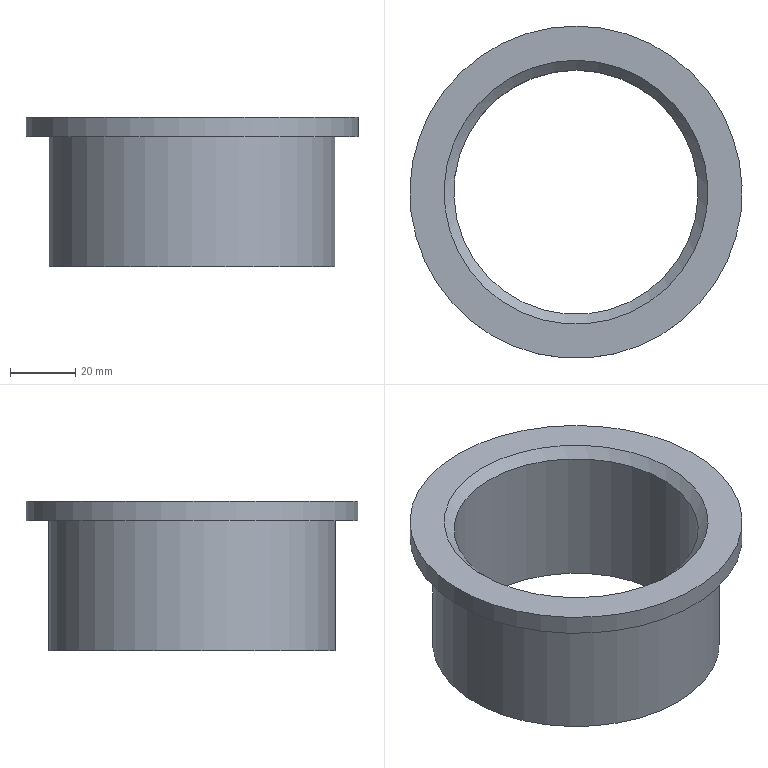Component | NX | 04__VALVE_SEAT__2 | 1 solid | 7 faces | box 102 x 102 x 46 mm | volume 88002 mm3 | cylinder 3 | plane 3 | cone 1 | commonest cylinder face diameters 75 x1 88 x1 102 x1
STEP:
#1=CARTESIAN_POINT('',(0.,0.,0.));
#2=DIRECTION('',(0.,0.,1.));
#3=DIRECTION('',(1.,0.,0.));
#4=AXIS2_PLACEMENT_3D('',#1,#2,#3);
#5=CARTESIAN_POINT('',(-6.375,36.231,610.));
#6=VERTEX_POINT('',#5);
#7=CARTESIAN_POINT('',(-6.375,-1.269,610.));
#8=DIRECTION('',(0.,0.,-1.));
#9=DIRECTION('',(-0.,1.,0.));
#10=AXIS2_PLACEMENT_3D('',#7,#8,#9);
#11=CIRCLE('',#10,37.5);
#12=CARTESIAN_POINT('',(-6.375,-1.269,610.));
#13=DIRECTION('',(0.,0.,-1.));
#14=DIRECTION('',(-0.,1.,0.));
#15=AXIS2_PLACEMENT_3D('',#12,#13,#14);
#16=CYLINDRICAL_SURFACE('',#15,37.5);
#17=CARTESIAN_POINT('',(0.,0.));
#18=DIRECTION('',(1.,0.));
#19=VECTOR('',#18,1.);
#20=LINE('',#17,#19);
#21=(GEOMETRIC_REPRESENTATION_CONTEXT(2)PARAMETRIC_REPRESENTATION_CONTEXT()REPRESENTATION_CONTEXT('',''));
#22=DEFINITIONAL_REPRESENTATION('',(#20),#21);
#23=PCURVE('',#16,#22);
#24=CARTESIAN_POINT('',(31.125,-1.269,610.));
#25=DIRECTION('',(0.,0.,-1.));
#26=DIRECTION('',(-0.,1.,0.));
#27=AXIS2_PLACEMENT_3D('',#24,#25,#26);
#28=PLANE('',#27);
#29=CARTESIAN_POINT('',(-0.,-37.5));
#30=DIRECTION('',(1.,-0.));
#31=AXIS2_PLACEMENT_2D('',#29,#30);
#32=CIRCLE('',#31,37.5);
#33=(GEOMETRIC_REPRESENTATION_CONTEXT(2)PARAMETRIC_REPRESENTATION_CONTEXT()REPRESENTATION_CONTEXT('',''));
#34=DEFINITIONAL_REPRESENTATION('',(#32),#33);
#35=PCURVE('',#28,#34);
#36=SURFACE_CURVE('',#11,(#23,#35),.PCURVE_S1.);
#37=EDGE_CURVE('',#6,#6,#36,.T.);
#38=ORIENTED_EDGE('',*,*,#37,.F.);
#39=CARTESIAN_POINT('',(-6.375,36.231,653.));
#40=VERTEX_POINT('',#39);
#41=CARTESIAN_POINT('',(-6.375,36.231,653.));
#42=CARTESIAN_POINT('',(-6.375,36.231,610.));
#43=B_SPLINE_CURVE_WITH_KNOTS('',1,(#41,#42),.UNSPECIFIED.,.F.,.F.,(2,2),(-43.,0.),.PIECEWISE_BEZIER_KNOTS.);
#44=CARTESIAN_POINT('',(0.,0.));
#45=DIRECTION('',(0.,1.));
#46=VECTOR('',#45,1.);
#47=LINE('',#44,#46);
#48=(GEOMETRIC_REPRESENTATION_CONTEXT(2)PARAMETRIC_REPRESENTATION_CONTEXT()REPRESENTATION_CONTEXT('',''));
#49=DEFINITIONAL_REPRESENTATION('',(#47),#48);
#50=PCURVE('',#16,#49);
#51=CARTESIAN_POINT('',(6.283,0.));
#52=DIRECTION('',(0.,1.));
#53=VECTOR('',#52,1.);
#54=LINE('',#51,#53);
#55=(GEOMETRIC_REPRESENTATION_CONTEXT(2)PARAMETRIC_REPRESENTATION_CONTEXT()REPRESENTATION_CONTEXT('',''));
#56=DEFINITIONAL_REPRESENTATION('',(#54),#55);
#57=PCURVE('',#16,#56);
#58=SEAM_CURVE('',#43,(#50,#57),.PCURVE_S1.);
#59=EDGE_CURVE('',#40,#6,#58,.T.);
#60=ORIENTED_EDGE('',*,*,#59,.F.);
#61=CARTESIAN_POINT('',(-6.375,-1.269,653.));
#62=DIRECTION('',(0.,0.,-1.));
#63=DIRECTION('',(-0.,1.,0.));
#64=AXIS2_PLACEMENT_3D('',#61,#62,#63);
#65=CIRCLE('',#64,37.5);
#66=CARTESIAN_POINT('',(0.,-43.));
#67=DIRECTION('',(1.,0.));
#68=VECTOR('',#67,1.);
#69=LINE('',#66,#68);
#70=(GEOMETRIC_REPRESENTATION_CONTEXT(2)PARAMETRIC_REPRESENTATION_CONTEXT()REPRESENTATION_CONTEXT('',''));
#71=DEFINITIONAL_REPRESENTATION('',(#69),#70);
#72=PCURVE('',#16,#71);
#73=CARTESIAN_POINT('',(-6.375,-1.269,656.));
#74=DIRECTION('',(0.,0.,1.));
#75=DIRECTION('',(0.,-1.,0.));
#76=AXIS2_PLACEMENT_3D('',#73,#74,#75);
#77=CONICAL_SURFACE('',#76,40.5,0.7854);
#78=CARTESIAN_POINT('',(9.425,-3.));
#79=DIRECTION('',(-1.,0.));
#80=VECTOR('',#79,1.);
#81=LINE('',#78,#80);
#82=(GEOMETRIC_REPRESENTATION_CONTEXT(2)PARAMETRIC_REPRESENTATION_CONTEXT()REPRESENTATION_CONTEXT('',''));
#83=DEFINITIONAL_REPRESENTATION('',(#81),#82);
#84=PCURVE('',#77,#83);
#85=SURFACE_CURVE('',#65,(#72,#84),.PCURVE_S1.);
#86=EDGE_CURVE('',#40,#40,#85,.T.);
#87=ORIENTED_EDGE('',*,*,#86,.T.);
#88=ORIENTED_EDGE('',*,*,#59,.T.);
#89=EDGE_LOOP('',(#38,#60,#87,#88));
#90=FACE_BOUND('',#89,.F.);
#91=ADVANCED_FACE('',(#90),#16,.F.);
#92=CARTESIAN_POINT('',(-6.375,42.731,610.));
#93=VERTEX_POINT('',#92);
#94=CARTESIAN_POINT('',(-6.375,-1.269,610.));
#95=DIRECTION('',(0.,0.,-1.));
#96=DIRECTION('',(-0.,1.,0.));
#97=AXIS2_PLACEMENT_3D('',#94,#95,#96);
#98=CIRCLE('',#97,44.);
#99=CARTESIAN_POINT('',(-0.,-37.5));
#100=DIRECTION('',(1.,0.));
#101=AXIS2_PLACEMENT_2D('',#99,#100);
#102=CIRCLE('',#101,44.);
#103=(GEOMETRIC_REPRESENTATION_CONTEXT(2)PARAMETRIC_REPRESENTATION_CONTEXT()REPRESENTATION_CONTEXT('',''));
#104=DEFINITIONAL_REPRESENTATION('',(#102),#103);
#105=PCURVE('',#28,#104);
#106=CARTESIAN_POINT('',(-6.375,-1.269,610.));
#107=DIRECTION('',(0.,0.,-1.));
#108=DIRECTION('',(-0.,1.,0.));
#109=AXIS2_PLACEMENT_3D('',#106,#107,#108);
#110=CYLINDRICAL_SURFACE('',#109,44.);
#111=CARTESIAN_POINT('',(0.,0.));
#112=DIRECTION('',(1.,0.));
#113=VECTOR('',#112,1.);
#114=LINE('',#111,#113);
#115=(GEOMETRIC_REPRESENTATION_CONTEXT(2)PARAMETRIC_REPRESENTATION_CONTEXT()REPRESENTATION_CONTEXT('',''));
#116=DEFINITIONAL_REPRESENTATION('',(#114),#115);
#117=PCURVE('',#110,#116);
#118=SURFACE_CURVE('',#98,(#105,#117),.PCURVE_S1.);
#119=EDGE_CURVE('',#93,#93,#118,.T.);
#120=ORIENTED_EDGE('',*,*,#119,.T.);
#121=EDGE_LOOP('',(#120));
#122=FACE_BOUND('',#121,.T.);
#123=ORIENTED_EDGE('',*,*,#37,.F.);
#124=EDGE_LOOP('',(#123));
#125=FACE_BOUND('',#124,.T.);
#126=ADVANCED_FACE('',(#122,#125),#28,.T.);
#127=CARTESIAN_POINT('',(-6.375,42.731,650.));
#128=VERTEX_POINT('',#127);
#129=CARTESIAN_POINT('',(-6.375,-1.269,650.));
#130=DIRECTION('',(0.,0.,-1.));
#131=DIRECTION('',(-0.,1.,0.));
#132=AXIS2_PLACEMENT_3D('',#129,#130,#131);
#133=CIRCLE('',#132,44.);
#134=CARTESIAN_POINT('',(0.,-40.));
#135=DIRECTION('',(1.,0.));
#136=VECTOR('',#135,1.);
#137=LINE('',#134,#136);
#138=(GEOMETRIC_REPRESENTATION_CONTEXT(2)PARAMETRIC_REPRESENTATION_CONTEXT()REPRESENTATION_CONTEXT('',''));
#139=DEFINITIONAL_REPRESENTATION('',(#137),#138);
#140=PCURVE('',#110,#139);
#141=CARTESIAN_POINT('',(37.625,-1.269,650.));
#142=DIRECTION('',(0.,0.,-1.));
#143=DIRECTION('',(-0.,1.,0.));
#144=AXIS2_PLACEMENT_3D('',#141,#142,#143);
#145=PLANE('',#144);
#146=CARTESIAN_POINT('',(0.,-44.));
#147=DIRECTION('',(1.,0.));
#148=AXIS2_PLACEMENT_2D('',#146,#147);
#149=CIRCLE('',#148,44.);
#150=(GEOMETRIC_REPRESENTATION_CONTEXT(2)PARAMETRIC_REPRESENTATION_CONTEXT()REPRESENTATION_CONTEXT('',''));
#151=DEFINITIONAL_REPRESENTATION('',(#149),#150);
#152=PCURVE('',#145,#151);
#153=SURFACE_CURVE('',#133,(#140,#152),.PCURVE_S1.);
#154=EDGE_CURVE('',#128,#128,#153,.T.);
#155=ORIENTED_EDGE('',*,*,#154,.T.);
#156=CARTESIAN_POINT('',(-6.375,42.731,650.));
#157=CARTESIAN_POINT('',(-6.375,42.731,610.));
#158=B_SPLINE_CURVE_WITH_KNOTS('',1,(#156,#157),.UNSPECIFIED.,.F.,.F.,(2,2),(-40.,0.),.PIECEWISE_BEZIER_KNOTS.);
#159=CARTESIAN_POINT('',(6.283,0.));
#160=DIRECTION('',(0.,1.));
#161=VECTOR('',#160,1.);
#162=LINE('',#159,#161);
#163=(GEOMETRIC_REPRESENTATION_CONTEXT(2)PARAMETRIC_REPRESENTATION_CONTEXT()REPRESENTATION_CONTEXT('',''));
#164=DEFINITIONAL_REPRESENTATION('',(#162),#163);
#165=PCURVE('',#110,#164);
#166=CARTESIAN_POINT('',(0.,0.));
#167=DIRECTION('',(0.,1.));
#168=VECTOR('',#167,1.);
#169=LINE('',#166,#168);
#170=(GEOMETRIC_REPRESENTATION_CONTEXT(2)PARAMETRIC_REPRESENTATION_CONTEXT()REPRESENTATION_CONTEXT('',''));
#171=DEFINITIONAL_REPRESENTATION('',(#169),#170);
#172=PCURVE('',#110,#171);
#173=SEAM_CURVE('',#158,(#165,#172),.PCURVE_S1.);
#174=EDGE_CURVE('',#128,#93,#173,.T.);
#175=ORIENTED_EDGE('',*,*,#174,.T.);
#176=ORIENTED_EDGE('',*,*,#119,.F.);
#177=ORIENTED_EDGE('',*,*,#174,.F.);
#178=EDGE_LOOP('',(#155,#175,#176,#177));
#179=FACE_BOUND('',#178,.T.);
#180=ADVANCED_FACE('',(#179),#110,.T.);
#181=CARTESIAN_POINT('',(-6.375,49.731,650.));
#182=VERTEX_POINT('',#181);
#183=CARTESIAN_POINT('',(-6.375,-1.269,650.));
#184=DIRECTION('',(0.,0.,-1.));
#185=DIRECTION('',(-0.,1.,0.));
#186=AXIS2_PLACEMENT_3D('',#183,#184,#185);
#187=CIRCLE('',#186,51.);
#188=CARTESIAN_POINT('',(0.,-44.));
#189=DIRECTION('',(1.,-0.));
#190=AXIS2_PLACEMENT_2D('',#188,#189);
#191=CIRCLE('',#190,51.);
#192=(GEOMETRIC_REPRESENTATION_CONTEXT(2)PARAMETRIC_REPRESENTATION_CONTEXT()REPRESENTATION_CONTEXT('',''));
#193=DEFINITIONAL_REPRESENTATION('',(#191),#192);
#194=PCURVE('',#145,#193);
#195=CARTESIAN_POINT('',(-6.375,-1.269,610.));
#196=DIRECTION('',(0.,0.,-1.));
#197=DIRECTION('',(-0.,1.,0.));
#198=AXIS2_PLACEMENT_3D('',#195,#196,#197);
#199=CYLINDRICAL_SURFACE('',#198,51.);
#200=CARTESIAN_POINT('',(0.,-40.));
#201=DIRECTION('',(1.,0.));
#202=VECTOR('',#201,1.);
#203=LINE('',#200,#202);
#204=(GEOMETRIC_REPRESENTATION_CONTEXT(2)PARAMETRIC_REPRESENTATION_CONTEXT()REPRESENTATION_CONTEXT('',''));
#205=DEFINITIONAL_REPRESENTATION('',(#203),#204);
#206=PCURVE('',#199,#205);
#207=SURFACE_CURVE('',#187,(#194,#206),.PCURVE_S1.);
#208=EDGE_CURVE('',#182,#182,#207,.T.);
#209=ORIENTED_EDGE('',*,*,#208,.T.);
#210=EDGE_LOOP('',(#209));
#211=FACE_BOUND('',#210,.T.);
#212=ORIENTED_EDGE('',*,*,#154,.F.);
#213=EDGE_LOOP('',(#212));
#214=FACE_BOUND('',#213,.T.);
#215=ADVANCED_FACE('',(#211,#214),#145,.T.);
#216=CARTESIAN_POINT('',(-6.375,49.731,656.));
#217=VERTEX_POINT('',#216);
#218=CARTESIAN_POINT('',(-6.375,-1.269,656.));
#219=DIRECTION('',(0.,0.,-1.));
#220=DIRECTION('',(-0.,1.,0.));
#221=AXIS2_PLACEMENT_3D('',#218,#219,#220);
#222=CIRCLE('',#221,51.);
#223=CARTESIAN_POINT('',(0.,-46.));
#224=DIRECTION('',(1.,0.));
#225=VECTOR('',#224,1.);
#226=LINE('',#223,#225);
#227=(GEOMETRIC_REPRESENTATION_CONTEXT(2)PARAMETRIC_REPRESENTATION_CONTEXT()REPRESENTATION_CONTEXT('',''));
#228=DEFINITIONAL_REPRESENTATION('',(#226),#227);
#229=PCURVE('',#199,#228);
#230=CARTESIAN_POINT('',(44.625,-1.269,656.));
#231=DIRECTION('',(0.,0.,1.));
#232=DIRECTION('',(0.,-1.,0.));
#233=AXIS2_PLACEMENT_3D('',#230,#231,#232);
#234=PLANE('',#233);
#235=CARTESIAN_POINT('',(-51.,-51.));
#236=CARTESIAN_POINT('',(-51.,37.335));
#237=CARTESIAN_POINT('',(25.5,-6.833));
#238=CARTESIAN_POINT('',(102.,-51.));
#239=CARTESIAN_POINT('',(25.5,-95.167));
#240=CARTESIAN_POINT('',(-51.,-139.335));
#241=CARTESIAN_POINT('',(-51.,-51.));
#242=(BOUNDED_CURVE()B_SPLINE_CURVE(2,(#235,#236,#237,#238,#239,#240,#241),.UNSPECIFIED.,.T.,.F.)B_SPLINE_CURVE_WITH_KNOTS((1,2,2,2,2,1),(-2.094,0.,2.094,4.189,6.283,8.378),.UNSPECIFIED.)CURVE()GEOMETRIC_REPRESENTATION_ITEM()RATIONAL_B_SPLINE_CURVE((1.,0.5,1.,0.5,1.,0.5,1.))REPRESENTATION_ITEM(''));
#243=(GEOMETRIC_REPRESENTATION_CONTEXT(2)PARAMETRIC_REPRESENTATION_CONTEXT()REPRESENTATION_CONTEXT('',''));
#244=DEFINITIONAL_REPRESENTATION('',(#242),#243);
#245=PCURVE('',#234,#244);
#246=SURFACE_CURVE('',#222,(#229,#245),.PCURVE_S1.);
#247=EDGE_CURVE('',#217,#217,#246,.T.);
#248=ORIENTED_EDGE('',*,*,#247,.T.);
#249=CARTESIAN_POINT('',(-6.375,49.731,656.));
#250=CARTESIAN_POINT('',(-6.375,49.731,650.));
#251=B_SPLINE_CURVE_WITH_KNOTS('',1,(#249,#250),.UNSPECIFIED.,.F.,.F.,(2,2),(-46.,-40.),.PIECEWISE_BEZIER_KNOTS.);
#252=CARTESIAN_POINT('',(6.283,0.));
#253=DIRECTION('',(0.,1.));
#254=VECTOR('',#253,1.);
#255=LINE('',#252,#254);
#256=(GEOMETRIC_REPRESENTATION_CONTEXT(2)PARAMETRIC_REPRESENTATION_CONTEXT()REPRESENTATION_CONTEXT('',''));
#257=DEFINITIONAL_REPRESENTATION('',(#255),#256);
#258=PCURVE('',#199,#257);
#259=CARTESIAN_POINT('',(0.,0.));
#260=DIRECTION('',(0.,1.));
#261=VECTOR('',#260,1.);
#262=LINE('',#259,#261);
#263=(GEOMETRIC_REPRESENTATION_CONTEXT(2)PARAMETRIC_REPRESENTATION_CONTEXT()REPRESENTATION_CONTEXT('',''));
#264=DEFINITIONAL_REPRESENTATION('',(#262),#263);
#265=PCURVE('',#199,#264);
#266=SEAM_CURVE('',#251,(#258,#265),.PCURVE_S1.);
#267=EDGE_CURVE('',#217,#182,#266,.T.);
#268=ORIENTED_EDGE('',*,*,#267,.T.);
#269=ORIENTED_EDGE('',*,*,#208,.F.);
#270=ORIENTED_EDGE('',*,*,#267,.F.);
#271=EDGE_LOOP('',(#248,#268,#269,#270));
#272=FACE_BOUND('',#271,.T.);
#273=ADVANCED_FACE('',(#272),#199,.T.);
#274=CARTESIAN_POINT('',(-6.375,39.231,656.));
#275=VERTEX_POINT('',#274);
#276=CARTESIAN_POINT('',(-6.375,-1.269,656.));
#277=DIRECTION('',(0.,0.,-1.));
#278=DIRECTION('',(-0.,1.,0.));
#279=AXIS2_PLACEMENT_3D('',#276,#277,#278);
#280=CIRCLE('',#279,40.5);
#281=CARTESIAN_POINT('',(-40.5,-51.));
#282=CARTESIAN_POINT('',(-40.5,19.148));
#283=CARTESIAN_POINT('',(20.25,-15.926));
#284=CARTESIAN_POINT('',(81.,-51.));
#285=CARTESIAN_POINT('',(20.25,-86.074));
#286=CARTESIAN_POINT('',(-40.5,-121.148));
#287=CARTESIAN_POINT('',(-40.5,-51.));
#288=(BOUNDED_CURVE()B_SPLINE_CURVE(2,(#281,#282,#283,#284,#285,#286,#287),.UNSPECIFIED.,.T.,.F.)B_SPLINE_CURVE_WITH_KNOTS((1,2,2,2,2,1),(-2.094,0.,2.094,4.189,6.283,8.378),.UNSPECIFIED.)CURVE()GEOMETRIC_REPRESENTATION_ITEM()RATIONAL_B_SPLINE_CURVE((1.,0.5,1.,0.5,1.,0.5,1.))REPRESENTATION_ITEM(''));
#289=(GEOMETRIC_REPRESENTATION_CONTEXT(2)PARAMETRIC_REPRESENTATION_CONTEXT()REPRESENTATION_CONTEXT('',''));
#290=DEFINITIONAL_REPRESENTATION('',(#288),#289);
#291=PCURVE('',#234,#290);
#292=CARTESIAN_POINT('',(9.425,0.));
#293=DIRECTION('',(-1.,0.));
#294=VECTOR('',#293,1.);
#295=LINE('',#292,#294);
#296=(GEOMETRIC_REPRESENTATION_CONTEXT(2)PARAMETRIC_REPRESENTATION_CONTEXT()REPRESENTATION_CONTEXT('',''));
#297=DEFINITIONAL_REPRESENTATION('',(#295),#296);
#298=PCURVE('',#77,#297);
#299=SURFACE_CURVE('',#280,(#291,#298),.PCURVE_S1.);
#300=EDGE_CURVE('',#275,#275,#299,.T.);
#301=ORIENTED_EDGE('',*,*,#300,.T.);
#302=EDGE_LOOP('',(#301));
#303=FACE_BOUND('',#302,.T.);
#304=ORIENTED_EDGE('',*,*,#247,.F.);
#305=EDGE_LOOP('',(#304));
#306=FACE_BOUND('',#305,.T.);
#307=ADVANCED_FACE('',(#303,#306),#234,.T.);
#308=ORIENTED_EDGE('',*,*,#86,.F.);
#309=CARTESIAN_POINT('',(-6.375,36.231,653.));
#310=CARTESIAN_POINT('',(-6.375,39.231,656.));
#311=B_SPLINE_CURVE_WITH_KNOTS('',1,(#309,#310),.UNSPECIFIED.,.F.,.F.,(2,2),(-4.243,0.),.PIECEWISE_BEZIER_KNOTS.);
#312=CARTESIAN_POINT('',(9.425,0.));
#313=DIRECTION('',(0.,1.));
#314=VECTOR('',#313,1.);
#315=LINE('',#312,#314);
#316=(GEOMETRIC_REPRESENTATION_CONTEXT(2)PARAMETRIC_REPRESENTATION_CONTEXT()REPRESENTATION_CONTEXT('',''));
#317=DEFINITIONAL_REPRESENTATION('',(#315),#316);
#318=PCURVE('',#77,#317);
#319=CARTESIAN_POINT('',(3.142,0.));
#320=DIRECTION('',(0.,1.));
#321=VECTOR('',#320,1.);
#322=LINE('',#319,#321);
#323=(GEOMETRIC_REPRESENTATION_CONTEXT(2)PARAMETRIC_REPRESENTATION_CONTEXT()REPRESENTATION_CONTEXT('',''));
#324=DEFINITIONAL_REPRESENTATION('',(#322),#323);
#325=PCURVE('',#77,#324);
#326=SEAM_CURVE('',#311,(#318,#325),.PCURVE_S1.);
#327=EDGE_CURVE('',#40,#275,#326,.T.);
#328=ORIENTED_EDGE('',*,*,#327,.T.);
#329=ORIENTED_EDGE('',*,*,#300,.T.);
#330=ORIENTED_EDGE('',*,*,#327,.F.);
#331=EDGE_LOOP('',(#308,#328,#329,#330));
#332=FACE_BOUND('',#331,.F.);
#333=ADVANCED_FACE('',(#332),#77,.F.);
#334=CLOSED_SHELL('',(#91,#126,#180,#215,#273,#307,#333));
#335=MANIFOLD_SOLID_BREP('',#334);
#336=(LENGTH_UNIT()NAMED_UNIT(*)SI_UNIT(.MILLI.,.METRE.));
#337=UNCERTAINTY_MEASURE_WITH_UNIT(LENGTH_MEASURE(0.00001),#336,'','');
#338=(NAMED_UNIT(*)PLANE_ANGLE_UNIT()SI_UNIT($,.RADIAN.));
#339=(NAMED_UNIT(*)SI_UNIT($,.STERADIAN.)SOLID_ANGLE_UNIT());
#340=(GEOMETRIC_REPRESENTATION_CONTEXT(3)GLOBAL_UNCERTAINTY_ASSIGNED_CONTEXT((#337))GLOBAL_UNIT_ASSIGNED_CONTEXT((#336,#338,#339))REPRESENTATION_CONTEXT('',''));
#341=ADVANCED_BREP_SHAPE_REPRESENTATION('',(#4,#335),#340);